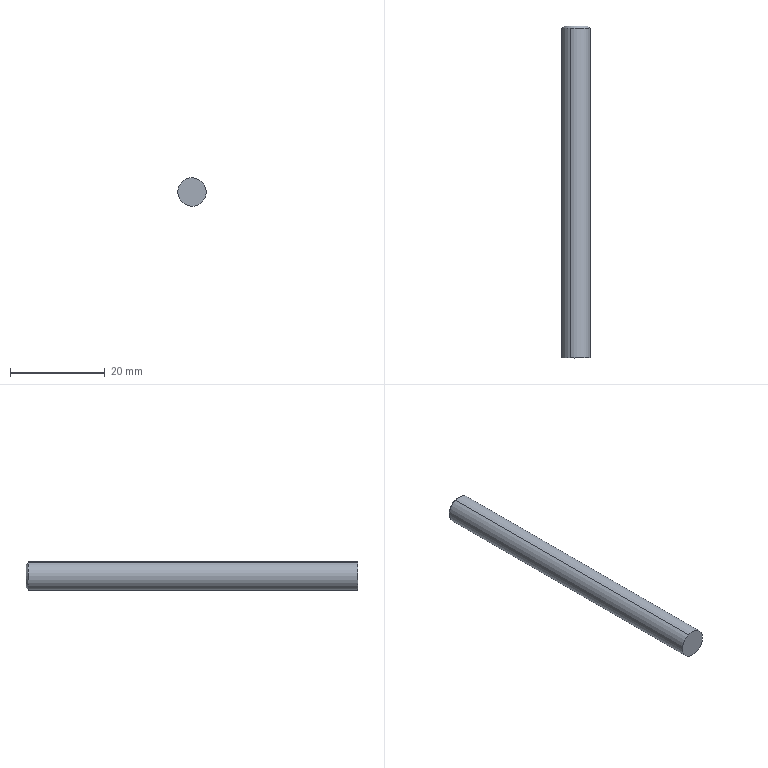Component | SolidWorks | GluePaperFeedingTensioningWheelAssembly-1_YX-04-116GluePaperFeedingTensioningWheelGuidePost-1 | 1 solid | 6 faces | box 6 x 70 x 6 mm | volume 1977 mm3 | cone 2 | cylinder 2 | plane 2 | commonest cylinder face diameters 6 x2 | material Hard Chrome Rod
build123d program:
from build123d import *


with BuildPart() as part:
    # Sketch1 → Revolve1 (revolve)
    with BuildSketch(Plane.XY, mode=Mode.PRIVATE) as revolve1_sk:
        Polygon((-35, 3), (-35, 0), (35, 0), (35, 2.5), (34.5, 3), align=None)
    revolve(revolve1_sk.sketch.rotate(Axis((-35, 0, 0), (1, 0, 0)), 270), axis=Axis((-35, 0, 0), (1, 0, 0)))


solid = part.part

# Placed as in the assembly
solid = solid.moved(Location((29.103, 6.262, 167), (0, 0, 90)))
STEP:
#1=CARTESIAN_POINT('',(1.108,1.624,6.666));
#2=VERTEX_POINT('',#1);
#3=CARTESIAN_POINT('',(1.183,1.624,6.484));
#4=VERTEX_POINT('',#3);
#5=CARTESIAN_POINT('',(1.146,1.624,6.575));
#6=DIRECTION('',(-0.,1.,0.));
#7=DIRECTION('',(-0.3818,0.,0.9242));
#8=AXIS2_PLACEMENT_3D('',#5,#6,#7);
#9=CIRCLE('',#8,0.09843);
#10=EDGE_CURVE('',#2,#4,#9,.T.);
#11=ORIENTED_EDGE('',*,*,#10,.F.);
#12=CARTESIAN_POINT('',(1.101,1.605,6.684));
#13=VERTEX_POINT('',#12);
#14=CARTESIAN_POINT('',(1.108,1.624,6.666));
#15=DIRECTION('',(-0.27,-0.7071,0.6535));
#16=VECTOR('',#15,39.37);
#17=LINE('',#14,#16);
#18=EDGE_CURVE('',#2,#13,#17,.T.);
#19=ORIENTED_EDGE('',*,*,#18,.T.);
#20=CARTESIAN_POINT('',(1.191,1.605,6.466));
#21=VERTEX_POINT('',#20);
#22=CARTESIAN_POINT('',(1.146,1.605,6.575));
#23=DIRECTION('',(-0.,1.,0.));
#24=DIRECTION('',(-0.3818,0.,0.9242));
#25=AXIS2_PLACEMENT_3D('',#22,#23,#24);
#26=CIRCLE('',#25,0.1181);
#27=EDGE_CURVE('',#13,#21,#26,.T.);
#28=ORIENTED_EDGE('',*,*,#27,.T.);
#29=CARTESIAN_POINT('',(1.183,1.624,6.484));
#30=DIRECTION('',(0.27,-0.7071,-0.6535));
#31=VECTOR('',#30,39.37);
#32=LINE('',#29,#31);
#33=EDGE_CURVE('',#4,#21,#32,.T.);
#34=ORIENTED_EDGE('',*,*,#33,.F.);
#35=EDGE_LOOP('',(#11,#19,#28,#34));
#36=FACE_OUTER_BOUND('',#35,.T.);
#37=CARTESIAN_POINT('',(1.146,1.624,6.575));
#38=DIRECTION('',(0.,-1.,-0.));
#39=DIRECTION('',(0.3818,0.,-0.9242));
#40=AXIS2_PLACEMENT_3D('',#37,#38,#39);
#41=CONICAL_SURFACE('',#40,0.09843,0.7854);
#42=ADVANCED_FACE('',(#36),#41,.T.);
#43=CARTESIAN_POINT('',(1.101,-1.131,6.684));
#44=VERTEX_POINT('',#43);
#45=CARTESIAN_POINT('',(1.191,-1.131,6.466));
#46=VERTEX_POINT('',#45);
#47=CARTESIAN_POINT('',(1.146,-1.131,6.575));
#48=DIRECTION('',(-0.,1.,0.));
#49=DIRECTION('',(-0.3818,0.,0.9242));
#50=AXIS2_PLACEMENT_3D('',#47,#48,#49);
#51=CIRCLE('',#50,0.1181);
#52=EDGE_CURVE('',#44,#46,#51,.T.);
#53=ORIENTED_EDGE('',*,*,#52,.T.);
#54=CARTESIAN_POINT('',(1.191,-1.131,6.466));
#55=DIRECTION('',(-0.,1.,0.));
#56=VECTOR('',#55,39.37);
#57=LINE('',#54,#56);
#58=EDGE_CURVE('',#46,#21,#57,.T.);
#59=ORIENTED_EDGE('',*,*,#58,.T.);
#60=ORIENTED_EDGE('',*,*,#27,.F.);
#61=CARTESIAN_POINT('',(1.101,-1.131,6.684));
#62=DIRECTION('',(-0.,1.,0.));
#63=VECTOR('',#62,39.37);
#64=LINE('',#61,#63);
#65=EDGE_CURVE('',#44,#13,#64,.T.);
#66=ORIENTED_EDGE('',*,*,#65,.F.);
#67=EDGE_LOOP('',(#53,#59,#60,#66));
#68=FACE_OUTER_BOUND('',#67,.T.);
#69=CARTESIAN_POINT('',(1.146,-1.131,6.575));
#70=DIRECTION('',(-0.,1.,0.));
#71=DIRECTION('',(-0.3818,0.,0.9242));
#72=AXIS2_PLACEMENT_3D('',#69,#70,#71);
#73=CYLINDRICAL_SURFACE('',#72,0.1181);
#74=ADVANCED_FACE('',(#68),#73,.T.);
#75=ORIENTED_EDGE('',*,*,#58,.F.);
#76=CARTESIAN_POINT('',(1.146,-1.131,6.575));
#77=DIRECTION('',(-0.,1.,0.));
#78=DIRECTION('',(-0.3818,0.,0.9242));
#79=AXIS2_PLACEMENT_3D('',#76,#77,#78);
#80=CIRCLE('',#79,0.1181);
#81=EDGE_CURVE('',#46,#44,#80,.T.);
#82=ORIENTED_EDGE('',*,*,#81,.T.);
#83=ORIENTED_EDGE('',*,*,#65,.T.);
#84=CARTESIAN_POINT('',(1.146,1.605,6.575));
#85=DIRECTION('',(-0.,1.,0.));
#86=DIRECTION('',(-0.3818,0.,0.9242));
#87=AXIS2_PLACEMENT_3D('',#84,#85,#86);
#88=CIRCLE('',#87,0.1181);
#89=EDGE_CURVE('',#21,#13,#88,.T.);
#90=ORIENTED_EDGE('',*,*,#89,.F.);
#91=EDGE_LOOP('',(#75,#82,#83,#90));
#92=FACE_OUTER_BOUND('',#91,.T.);
#93=CARTESIAN_POINT('',(1.146,-1.131,6.575));
#94=DIRECTION('',(-0.,1.,0.));
#95=DIRECTION('',(-0.3818,0.,0.9242));
#96=AXIS2_PLACEMENT_3D('',#93,#94,#95);
#97=CYLINDRICAL_SURFACE('',#96,0.1181);
#98=ADVANCED_FACE('',(#92),#97,.T.);
#99=ORIENTED_EDGE('',*,*,#52,.F.);
#100=ORIENTED_EDGE('',*,*,#81,.F.);
#101=EDGE_LOOP('',(#99,#100));
#102=FACE_OUTER_BOUND('',#101,.T.);
#103=CARTESIAN_POINT('',(1.255,-1.131,6.62));
#104=DIRECTION('',(0.,-1.,-0.));
#105=DIRECTION('',(0.3818,0.,-0.9242));
#106=AXIS2_PLACEMENT_3D('',#103,#104,#105);
#107=PLANE('',#106);
#108=ADVANCED_FACE('',(#102),#107,.T.);
#109=CARTESIAN_POINT('',(1.146,1.624,6.575));
#110=DIRECTION('',(-0.,1.,0.));
#111=DIRECTION('',(-0.3818,0.,0.9242));
#112=AXIS2_PLACEMENT_3D('',#109,#110,#111);
#113=CIRCLE('',#112,0.09843);
#114=EDGE_CURVE('',#4,#2,#113,.T.);
#115=ORIENTED_EDGE('',*,*,#114,.T.);
#116=ORIENTED_EDGE('',*,*,#10,.T.);
#117=EDGE_LOOP('',(#115,#116));
#118=FACE_OUTER_BOUND('',#117,.T.);
#119=CARTESIAN_POINT('',(1.146,1.624,6.575));
#120=DIRECTION('',(-0.,1.,0.));
#121=DIRECTION('',(-0.3818,-0.,0.9242));
#122=AXIS2_PLACEMENT_3D('',#119,#120,#121);
#123=PLANE('',#122);
#124=ADVANCED_FACE('',(#118),#123,.T.);
#125=ORIENTED_EDGE('',*,*,#18,.F.);
#126=ORIENTED_EDGE('',*,*,#114,.F.);
#127=ORIENTED_EDGE('',*,*,#33,.T.);
#128=ORIENTED_EDGE('',*,*,#89,.T.);
#129=EDGE_LOOP('',(#125,#126,#127,#128));
#130=FACE_OUTER_BOUND('',#129,.T.);
#131=CARTESIAN_POINT('',(1.146,1.624,6.575));
#132=DIRECTION('',(0.,-1.,-0.));
#133=DIRECTION('',(0.3818,0.,-0.9242));
#134=AXIS2_PLACEMENT_3D('',#131,#132,#133);
#135=CONICAL_SURFACE('',#134,0.09843,0.7854);
#136=ADVANCED_FACE('',(#130),#135,.T.);
#137=CLOSED_SHELL('',(#42,#74,#98,#108,#124,#136));
#138=MANIFOLD_SOLID_BREP('',#137);
#139=CARTESIAN_POINT('',(0.,0.,0.));
#140=DIRECTION('',(0.,0.,1.));
#141=DIRECTION('',(1.,0.,0.));
#142=AXIS2_PLACEMENT_3D('',#139,#140,#141);
#143=(LENGTH_UNIT()NAMED_UNIT(*)SI_UNIT($,.METRE.));
#144=LENGTH_MEASURE_WITH_UNIT(LENGTH_MEASURE(0.0254),#143);
#145=DIMENSIONAL_EXPONENTS(1.,0.,0.,0.,0.,0.,0.);
#146=(CONVERSION_BASED_UNIT('',#144)LENGTH_UNIT()NAMED_UNIT(#145));
#147=UNCERTAINTY_MEASURE_WITH_UNIT(LENGTH_MEASURE(0.00001),#146,'','');
#148=(NAMED_UNIT(*)PLANE_ANGLE_UNIT()SI_UNIT($,.RADIAN.));
#149=(NAMED_UNIT(*)SI_UNIT($,.STERADIAN.)SOLID_ANGLE_UNIT());
#150=(GEOMETRIC_REPRESENTATION_CONTEXT(3)GLOBAL_UNCERTAINTY_ASSIGNED_CONTEXT((#147))GLOBAL_UNIT_ASSIGNED_CONTEXT((#146,#148,#149))REPRESENTATION_CONTEXT('',''));
#151=ADVANCED_BREP_SHAPE_REPRESENTATION('',(#138,#142),#150);
#152=COLOUR_RGB('',0.7922,0.8196,0.9333);
#153=FILL_AREA_STYLE_COLOUR('',#152);
#154=FILL_AREA_STYLE('',(#153));
#155=SURFACE_STYLE_FILL_AREA(#154);
#156=SURFACE_SIDE_STYLE('',(#155));
#157=SURFACE_STYLE_USAGE(.BOTH.,#156);
#158=PRESENTATION_STYLE_ASSIGNMENT((#157));
#159=STYLED_ITEM('',(#158),#138);
#160=(LENGTH_UNIT()NAMED_UNIT(*)SI_UNIT($,.METRE.));
#161=LENGTH_MEASURE_WITH_UNIT(LENGTH_MEASURE(0.0254),#160);
#162=DIMENSIONAL_EXPONENTS(1.,0.,0.,0.,0.,0.,0.);
#163=(CONVERSION_BASED_UNIT('',#161)LENGTH_UNIT()NAMED_UNIT(#162));
#164=UNCERTAINTY_MEASURE_WITH_UNIT(LENGTH_MEASURE(0.00001),#163,'','');
#165=(NAMED_UNIT(*)PLANE_ANGLE_UNIT()SI_UNIT($,.RADIAN.));
#166=(NAMED_UNIT(*)SI_UNIT($,.STERADIAN.)SOLID_ANGLE_UNIT());
#167=(GEOMETRIC_REPRESENTATION_CONTEXT(3)GLOBAL_UNCERTAINTY_ASSIGNED_CONTEXT((#164))GLOBAL_UNIT_ASSIGNED_CONTEXT((#163,#165,#166))REPRESENTATION_CONTEXT('',''));
#168=MECHANICAL_DESIGN_GEOMETRIC_PRESENTATION_REPRESENTATION('',(#159),#167);
#169=PRESENTATION_LAYER_ASSIGNMENT('','',(#159));